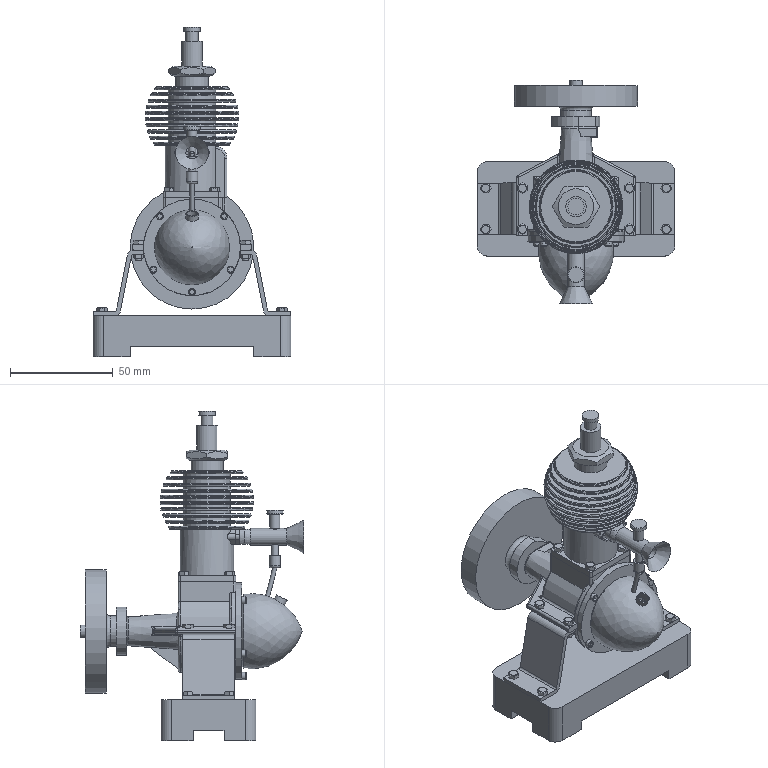Assembly | NX | mm | 40 component files | 40 solids | 841 faces | box 96 x 108.5 x 160.3 mm | volume 169682 mm3 | plane 422 | cylinder 253 | cone 73 | torus 48 | sphere 23 | spline 22 | commonest cylinder face diameters 2 x51 3 x38 0.5 x31 6 x14 2.5 x13 3.5 x9 23 x9 10 x8
Bill of materials:
unnamed part 1 | 1 |  | Thick flat disc with a central through hole and one straight flat cut on its outer edge (D-shaped outline).
unnamed part 2 | 1 |  | Large flat disc with a small cylindrical hub on one face and a small central through bore, possibly a wheel or knob blank.
unnamed part 3 | 5 |  | Cap-screw-like shape: cylindrical head with a hexagonal socket recess and a plain cylindrical shank with chamfered ends.
unnamed part 4 | 1 |  | Nail- or tack-like pin with a flat round head, a stepped cylindrical shank and a sharp conical point.
unnamed part 5 | 1 |  | Flanged cylindrical ring or cup: a thin circular flange with five evenly spaced bolt holes, plus a raised cylindrical collar that forms a large central recess.
unnamed part 6 | 1 |  | Long slender rod with a short hollow cylindrical collar at one end and a rounded opposite tip.
unnamed part 7 | 1 |  | Hollow tubular body with a conical flared funnel at one end, a transverse through hole in the tube wall, and a rectangular flange-like end block with small tabs.
unnamed part 8 | 1 |  | Piston-like cylindrical body with three circumferential grooves near the top, a raised rounded crown inclined to the axis, and a transverse through hole in the skirt.
unnamed part 9 | 1 |  | Rounded ogive or dome-shaped body ending in a cylindrical neck, with a small hollow cylindrical boss and a small hole on its curved surface.
unnamed part 10 | 1 |  | Stepped axisymmetric shaft with a hexagonal collar in the middle: a smaller stepped pin with a head-like end on one side and cylindrical spigots on the other.
unnamed part 11 | 1 |  | Tubular pin with a larger cylindrical head-like collar, an axial bore with a conical entry, and a transverse through hole in the smaller shank.
unnamed part 12 | 1 |  | Plain solid cylindrical pin with chamfered edges at both ends.
unnamed part 13 | 1 |  | Vertical cylindrical body with a stack of about ten thin circular fins around its upper portion, forming a rounded, roughly spherical outline. A domed top has a central through-hole. Below the fins is a plain cylindrical section with a rectangular side boss and a vertical side duct/boss, a square flange with corner holes, and a short cylindrical spigot under the flange.
unnamed part 14 | 1 |  | Thin flat rectangular plate with two equal circular through-holes positioned along its long axis near each end.
unnamed part 15 | 12 |  | Hex-head fastener-like part: a hexagonal head with chamfered top corners and a plain cylindrical shank with a chamfered end.
unnamed part 16 | 1 |  | Complex housing with a large cylindrical bore. One end has a circular flange with bolt holes and a smaller central hole in the end wall. On top is a square pad with corner holes and a circular opening with a notched recess. A tapered tubular boss sticks out sideways and ends in a small rectangular flange. Flat mounting lugs/flanges with holes extend from the sides.
unnamed part 17 | 4 |  | Hexagonal nut-like part with a large plain central through-hole and double-chamfered (curved-arc) corners on both faces. It is relatively thin compared with its width.
unnamed part 18 | 2 |  | Bent sheet-like Z-shaped bracket: two parallel flat flanges joined by an inclined web with rounded bends. Each flange has two through-holes.
unnamed part 19 | 1 |  | Rectangular block with rounded vertical corners and a flat top. Four small holes sit near the short ends. The underside has rectangular stepped cutouts/notches that leave foot-like portions.
unnamed part 20 | 1 |  | Link/rod-like part with two cylindrical ring ends of different diameters joined by a slender tapered beam. A shallow elongated recess runs along the beam face.
unnamed part 21 | 1 |  | Shaft with a semicircular/segment-shaped disc web near one end. A long main shaft with a stepped taper extends from one side. On the other side, a short offset pin with a circumferential groove extends from a rectangular arm.
Mates:
1. fix | base_plate 1 component
2. concentric | base_plate 1 edge | bracket 2 edge
3. concentric | base_plate 1 edge | bracket 1 edge
4. concentric | bracket 2 edge | cylinder_block 1 edge
5. parallel | cylinder_block 1 face | base_plate 1 face
6. parallel | bracket 2 face | base_plate 1 face
7. parallel | bracket 1 face | base_plate 1 face
8. concentric | cylinder_block 1 edge | piston_cylinder 1 arc
9. parallel | piston_cylinder 1 face | cylinder_block 1 face
10. concentric | cylinder_block 1 edge | flange 1 edge
11. concentric | cylinder_block 1 edge | flange 1 edge
12. touch align | cylinder_cap 1 face | flange 1 face
13. touch align | cylinder_cap 1 face | flange 1 face
14. concentric | cam 1 edge | cylinder_block 1 edge
15. center | crankshaft 1 face | crankshaft 1 face | cylinder_block 1 face
16. bond | cam 1 component | pulley 1 component | crankshaft 1 component
17. concentric | piston_cylinder 1 edge | air_cylinder 1 edge
18. parallel | air_cylinder 1 face | piston_cylinder 1 face
19. touch align | con_rod 1 face | crankshaft 1 face
20. center | con_rod 1 face | con_rod 1 face | piston_cylinder 1 face
21. touch align | con_rod 1 face | piston 1 face
22. center | con_rod 1 face | con_rod 1 face | piston 1 face
23. distance | piston 1 face | piston_cylinder 1 face
24. touch align | air_pump_part_01_11 1 face | air_cylinder 1 face
25. touch align | air_cylinder 1 face | air_pump_part_01_11 1 edge
26. concentric | air_pump_part_01_20 1 edge | air_pump_part_01_11 1 edge
27. concentric | air_pump_part_01_11 1 edge | air_pump_part_01_12 1 edge
28. fix | air_pump_part_01_12 1 component
29. concentric | air_pump_part_01_18 1 arc | cylinder_block 1 edge
30. parallel | air_pump_part_01_18 1 face | cylinder_block 1 face
31. concentric | piston_cylinder 1 edge | spark_plug 1 edge
32. concentric | piston_cylinder 1 edge | screw_M3X8 12 edge
33. parallel | screw_M3X8 12 face | piston_cylinder 1 face
34. concentric | piston_cylinder 1 edge | screw_M3X8 11 edge
35. parallel | screw_M3X8 11 face | piston_cylinder 1 face
36. concentric | piston_cylinder 1 edge | screw_M3X8 10 edge
37. parallel | screw_M3X8 10 face | piston_cylinder 1 face
38. concentric | piston_cylinder 1 edge | screw_M3X8 9 edge
39. parallel | screw_M3X8 9 face | piston_cylinder 1 face
40. concentric | cylinder_block 1 edge | screw_M3X8 8 edge
41. concentric | cylinder_block 1 edge | screw_M3X8 7 edge
42. parallel | screw_M3X8 7 face | cylinder_block 1 face
43. parallel | screw_M3X8 8 face | cylinder_block 1 face
44. concentric | cylinder_block 1 edge | screw_M3X8 6 edge
45. parallel | screw_M3X8 6 face | cylinder_block 1 face
46. concentric | cylinder_block 1 edge | screw_M3X8 5 edge
47. parallel | screw_M3X8 5 face | cylinder_block 1 face
48. concentric | bracket 2 edge | screw_M3X8 4 edge
49. parallel | screw_M3X8 4 face | bracket 2 face
50. concentric | bracket 2 edge | screw_M3X8 3 edge
51. parallel | screw_M3X8 3 face | bracket 2 face
52. concentric | bracket 1 edge | screw_M3X8 2 edge
53. parallel | screw_M3X8 2 face | bracket 1 face
54. concentric | bracket 1 edge | screw_M3X8 1 edge
55. parallel | screw_M3X8 1 face | bracket 1 face
56. parallel | nut_M3 4 face | bracket 1 face
57. parallel | nut_M3 3 face | nut_M3 4 face
58. parallel | nut_M3 2 face | bracket 2 face
59. parallel | nut_M3 1 face | bracket 2 face
60. concentric | flange 1 edge | screw_M2_5X5 5 arc
61. concentric | flange 1 edge | screw_M2_5X5 4 arc
62. concentric | screw_M2_5X5 3 arc | flange 1 edge
63. concentric | flange 1 edge | screw_M2_5X5 2 arc
64. concentric | flange 1 edge | screw_M2_5X5 1 arc
65. touch align | pin 1 face | piston 1 face
66. center | pin 1 face | pin 1 face | piston 1 face